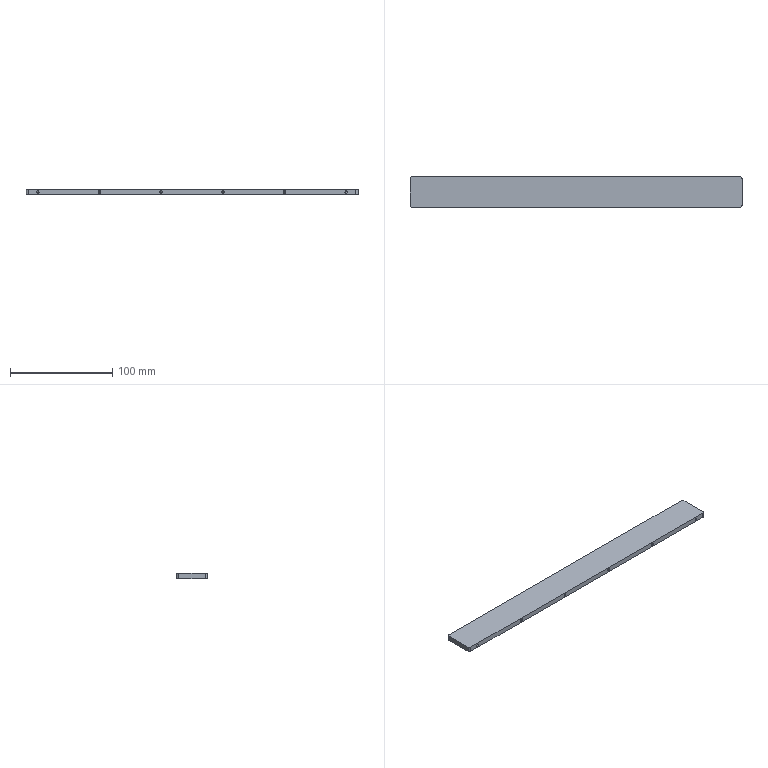CAM job | Mastercam | mm | 4 operations | part box 325 x 30 x 5
1. Contour (Ramp) | 4 - 4 平铣刀
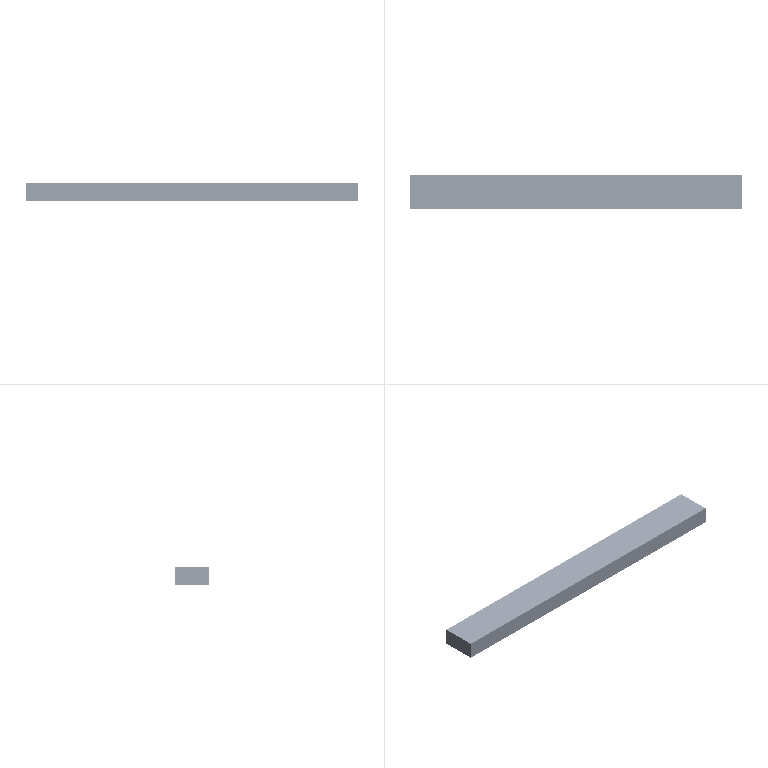2. Contour (2D) | 3 - 3 平铣刀
3. Contour (2D chamfer) | 5 - 4 倒角刀
4. Drill/Counterbore | 5 - 4 倒角刀